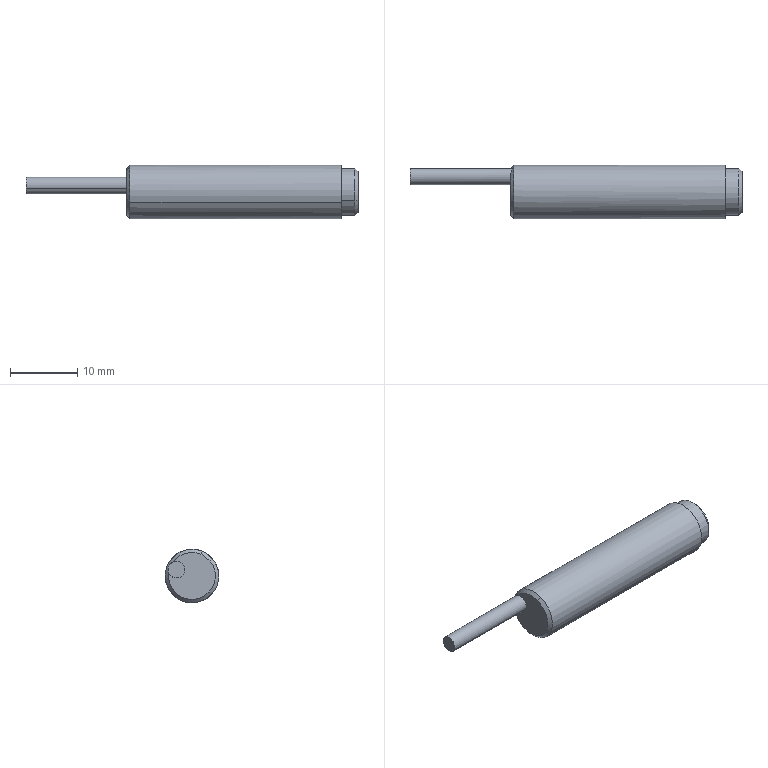Component | SolidWorks | PR8-2DN_1ProximitySwitch-1 | 1 solid | 14 faces | box 49.5 x 8 x 8 mm | volume 1773 mm3 | cylinder 6 | cone 4 | plane 4 | commonest cylinder face diameters 8 x2 7 x2 2.5 x2 | material 45#Steel
STEP:
#1=COLOUR_RGB('',0.7922,0.8196,0.9333);
#2=FILL_AREA_STYLE_COLOUR('',#1);
#3=FILL_AREA_STYLE('',(#2));
#4=SURFACE_STYLE_FILL_AREA(#3);
#5=SURFACE_SIDE_STYLE('',(#4));
#6=SURFACE_STYLE_USAGE(.BOTH.,#5);
#7=PRESENTATION_STYLE_ASSIGNMENT((#6));
#8=CARTESIAN_POINT('',(-0.2322,0.9159,6.515));
#9=VERTEX_POINT('',#8);
#10=CARTESIAN_POINT('',(-0.2322,1.207,6.635));
#11=VERTEX_POINT('',#10);
#12=CARTESIAN_POINT('',(-0.2322,1.061,6.575));
#13=DIRECTION('',(-1.,-0.,-0.));
#14=DIRECTION('',(0.,-0.9245,-0.3811));
#15=AXIS2_PLACEMENT_3D('',#12,#13,#14);
#16=CIRCLE('',#15,0.1575);
#17=EDGE_CURVE('',#9,#11,#16,.T.);
#18=ORIENTED_EDGE('',*,*,#17,.T.);
#19=CARTESIAN_POINT('',(-1.472,1.207,6.635));
#20=VERTEX_POINT('',#19);
#21=CARTESIAN_POINT('',(-0.2322,1.207,6.635));
#22=DIRECTION('',(-1.,-0.,-0.));
#23=VECTOR('',#22,39.37);
#24=LINE('',#21,#23);
#25=EDGE_CURVE('',#11,#20,#24,.T.);
#26=ORIENTED_EDGE('',*,*,#25,.T.);
#27=CARTESIAN_POINT('',(-1.472,1.001,6.72));
#28=VERTEX_POINT('',#27);
#29=CARTESIAN_POINT('',(-1.472,1.061,6.575));
#30=DIRECTION('',(1.,0.,0.));
#31=DIRECTION('',(0.,-0.9245,-0.3811));
#32=AXIS2_PLACEMENT_3D('',#29,#30,#31);
#33=CIRCLE('',#32,0.1575);
#34=EDGE_CURVE('',#20,#28,#33,.T.);
#35=ORIENTED_EDGE('',*,*,#34,.T.);
#36=CARTESIAN_POINT('',(-1.472,0.9159,6.515));
#37=VERTEX_POINT('',#36);
#38=CARTESIAN_POINT('',(-1.472,1.061,6.575));
#39=DIRECTION('',(1.,0.,0.));
#40=DIRECTION('',(0.,-0.9245,-0.3811));
#41=AXIS2_PLACEMENT_3D('',#38,#39,#40);
#42=CIRCLE('',#41,0.1575);
#43=EDGE_CURVE('',#28,#37,#42,.T.);
#44=ORIENTED_EDGE('',*,*,#43,.T.);
#45=CARTESIAN_POINT('',(-0.2322,0.9159,6.515));
#46=DIRECTION('',(-1.,-0.,-0.));
#47=VECTOR('',#46,39.37);
#48=LINE('',#45,#47);
#49=EDGE_CURVE('',#9,#37,#48,.T.);
#50=ORIENTED_EDGE('',*,*,#49,.F.);
#51=EDGE_LOOP('',(#18,#26,#35,#44,#50));
#52=FACE_OUTER_BOUND('',#51,.T.);
#53=CARTESIAN_POINT('',(-0.2322,1.061,6.575));
#54=DIRECTION('',(-1.,-0.,-0.));
#55=DIRECTION('',(0.,-0.9245,-0.3811));
#56=AXIS2_PLACEMENT_3D('',#53,#54,#55);
#57=CYLINDRICAL_SURFACE('',#56,0.1575);
#58=ADVANCED_FACE('',(#52),#57,.T.);
#59=CARTESIAN_POINT('',(-1.492,1.172,6.658));
#60=VERTEX_POINT('',#59);
#61=CARTESIAN_POINT('',(-1.492,1.009,6.702));
#62=VERTEX_POINT('',#61);
#63=CARTESIAN_POINT('',(-1.492,1.061,6.575));
#64=DIRECTION('',(1.,-0.,0.));
#65=DIRECTION('',(0.,0.3811,-0.9245));
#66=AXIS2_PLACEMENT_3D('',#63,#64,#65);
#67=CIRCLE('',#66,0.1378);
#68=EDGE_CURVE('',#60,#62,#67,.T.);
#69=ORIENTED_EDGE('',*,*,#68,.T.);
#70=CARTESIAN_POINT('',(-1.472,1.001,6.72));
#71=DIRECTION('',(0.7071,-0.2695,0.6537));
#72=VECTOR('',#71,39.37);
#73=LINE('',#70,#72);
#74=EDGE_CURVE('',#62,#28,#73,.T.);
#75=ORIENTED_EDGE('',*,*,#74,.T.);
#76=ORIENTED_EDGE('',*,*,#34,.F.);
#77=CARTESIAN_POINT('',(-1.472,1.122,6.429));
#78=VERTEX_POINT('',#77);
#79=CARTESIAN_POINT('',(-1.472,1.061,6.575));
#80=DIRECTION('',(1.,0.,0.));
#81=DIRECTION('',(0.,-0.9245,-0.3811));
#82=AXIS2_PLACEMENT_3D('',#79,#80,#81);
#83=CIRCLE('',#82,0.1575);
#84=EDGE_CURVE('',#78,#20,#83,.T.);
#85=ORIENTED_EDGE('',*,*,#84,.F.);
#86=CARTESIAN_POINT('',(-1.492,1.114,6.447));
#87=VERTEX_POINT('',#86);
#88=CARTESIAN_POINT('',(-1.472,1.122,6.429));
#89=DIRECTION('',(0.7071,0.2695,-0.6537));
#90=VECTOR('',#89,39.37);
#91=LINE('',#88,#90);
#92=EDGE_CURVE('',#87,#78,#91,.T.);
#93=ORIENTED_EDGE('',*,*,#92,.F.);
#94=CARTESIAN_POINT('',(-1.492,1.198,6.594));
#95=VERTEX_POINT('',#94);
#96=CARTESIAN_POINT('',(-1.492,1.061,6.575));
#97=DIRECTION('',(1.,-0.,0.));
#98=DIRECTION('',(0.,0.3811,-0.9245));
#99=AXIS2_PLACEMENT_3D('',#96,#97,#98);
#100=CIRCLE('',#99,0.1378);
#101=EDGE_CURVE('',#87,#95,#100,.T.);
#102=ORIENTED_EDGE('',*,*,#101,.T.);
#103=CARTESIAN_POINT('',(-1.482,1.198,6.631));
#104=VERTEX_POINT('',#103);
#105=CARTESIAN_POINT('',(-1.492,1.198,6.594));
#106=CARTESIAN_POINT('',(-1.491,1.199,6.596));
#107=CARTESIAN_POINT('',(-1.489,1.2,6.599));
#108=CARTESIAN_POINT('',(-1.487,1.201,6.605));
#109=CARTESIAN_POINT('',(-1.486,1.202,6.609));
#110=CARTESIAN_POINT('',(-1.484,1.202,6.615));
#111=CARTESIAN_POINT('',(-1.483,1.201,6.618));
#112=CARTESIAN_POINT('',(-1.482,1.2,6.625));
#113=CARTESIAN_POINT('',(-1.482,1.199,6.628));
#114=CARTESIAN_POINT('',(-1.482,1.198,6.631));
#115=B_SPLINE_CURVE_WITH_KNOTS('',3,(#105,#106,#107,#108,#109,#110,#111,#112,#113,#114),.UNSPECIFIED.,.F.,.F.,(4,2,2,2,4),(0.,0.0002535,0.000507,0.0007605,0.001014),.UNSPECIFIED.);
#116=EDGE_CURVE('',#95,#104,#115,.T.);
#117=ORIENTED_EDGE('',*,*,#116,.T.);
#118=CARTESIAN_POINT('',(-1.482,1.198,6.631));
#119=CARTESIAN_POINT('',(-1.482,1.197,6.634));
#120=CARTESIAN_POINT('',(-1.482,1.195,6.637));
#121=CARTESIAN_POINT('',(-1.483,1.191,6.643));
#122=CARTESIAN_POINT('',(-1.484,1.189,6.645));
#123=CARTESIAN_POINT('',(-1.487,1.182,6.652));
#124=CARTESIAN_POINT('',(-1.489,1.177,6.655));
#125=CARTESIAN_POINT('',(-1.492,1.172,6.658));
#126=B_SPLINE_CURVE_WITH_KNOTS('',3,(#118,#119,#120,#121,#122,#123,#124,#125),.UNSPECIFIED.,.F.,.F.,(4,2,2,4),(0.001014,0.001267,0.001519,0.002025),.UNSPECIFIED.);
#127=EDGE_CURVE('',#104,#60,#126,.T.);
#128=ORIENTED_EDGE('',*,*,#127,.T.);
#129=EDGE_LOOP('',(#69,#75,#76,#85,#93,#102,#117,#128));
#130=FACE_OUTER_BOUND('',#129,.T.);
#131=CARTESIAN_POINT('',(-1.472,1.061,6.575));
#132=DIRECTION('',(1.,-0.,0.));
#133=DIRECTION('',(0.,0.3811,-0.9245));
#134=AXIS2_PLACEMENT_3D('',#131,#132,#133);
#135=CONICAL_SURFACE('',#134,0.1575,0.7854);
#136=ADVANCED_FACE('',(#130),#135,.T.);
#137=CARTESIAN_POINT('',(-0.2322,1.189,6.627));
#138=VERTEX_POINT('',#137);
#139=CARTESIAN_POINT('',(-0.2322,0.9341,6.522));
#140=VERTEX_POINT('',#139);
#141=CARTESIAN_POINT('',(-0.2322,1.061,6.575));
#142=DIRECTION('',(1.,0.,0.));
#143=DIRECTION('',(0.,0.9245,0.3811));
#144=AXIS2_PLACEMENT_3D('',#141,#142,#143);
#145=CIRCLE('',#144,0.1378);
#146=EDGE_CURVE('',#138,#140,#145,.T.);
#147=ORIENTED_EDGE('',*,*,#146,.T.);
#148=CARTESIAN_POINT('',(-0.1534,0.9341,6.522));
#149=VERTEX_POINT('',#148);
#150=CARTESIAN_POINT('',(-0.2322,0.9341,6.522));
#151=DIRECTION('',(1.,0.,0.));
#152=VECTOR('',#151,39.37);
#153=LINE('',#150,#152);
#154=EDGE_CURVE('',#140,#149,#153,.T.);
#155=ORIENTED_EDGE('',*,*,#154,.T.);
#156=CARTESIAN_POINT('',(-0.1534,1.189,6.627));
#157=VERTEX_POINT('',#156);
#158=CARTESIAN_POINT('',(-0.1534,1.061,6.575));
#159=DIRECTION('',(-1.,-0.,-0.));
#160=DIRECTION('',(-0.,0.9245,0.3811));
#161=AXIS2_PLACEMENT_3D('',#158,#159,#160);
#162=CIRCLE('',#161,0.1378);
#163=EDGE_CURVE('',#149,#157,#162,.T.);
#164=ORIENTED_EDGE('',*,*,#163,.T.);
#165=CARTESIAN_POINT('',(-0.2322,1.189,6.627));
#166=DIRECTION('',(1.,0.,0.));
#167=VECTOR('',#166,39.37);
#168=LINE('',#165,#167);
#169=EDGE_CURVE('',#138,#157,#168,.T.);
#170=ORIENTED_EDGE('',*,*,#169,.F.);
#171=EDGE_LOOP('',(#147,#155,#164,#170));
#172=FACE_OUTER_BOUND('',#171,.T.);
#173=CARTESIAN_POINT('',(-0.2322,1.061,6.575));
#174=DIRECTION('',(1.,0.,0.));
#175=DIRECTION('',(0.,0.9245,0.3811));
#176=AXIS2_PLACEMENT_3D('',#173,#174,#175);
#177=CYLINDRICAL_SURFACE('',#176,0.1378);
#178=ADVANCED_FACE('',(#172),#177,.T.);
#179=ORIENTED_EDGE('',*,*,#127,.F.);
#180=CARTESIAN_POINT('',(-2.083,1.198,6.631));
#181=VERTEX_POINT('',#180);
#182=CARTESIAN_POINT('',(-1.492,1.198,6.631));
#183=DIRECTION('',(-1.,-0.,-0.));
#184=VECTOR('',#183,39.37);
#185=LINE('',#182,#184);
#186=EDGE_CURVE('',#104,#181,#185,.T.);
#187=ORIENTED_EDGE('',*,*,#186,.T.);
#188=CARTESIAN_POINT('',(-2.083,1.107,6.594));
#189=VERTEX_POINT('',#188);
#190=CARTESIAN_POINT('',(-2.083,1.152,6.612));
#191=DIRECTION('',(1.,0.,0.));
#192=DIRECTION('',(0.,-0.9245,-0.3811));
#193=AXIS2_PLACEMENT_3D('',#190,#191,#192);
#194=CIRCLE('',#193,0.04921);
#195=EDGE_CURVE('',#181,#189,#194,.T.);
#196=ORIENTED_EDGE('',*,*,#195,.T.);
#197=CARTESIAN_POINT('',(-1.492,1.107,6.594));
#198=VERTEX_POINT('',#197);
#199=CARTESIAN_POINT('',(-1.492,1.107,6.594));
#200=DIRECTION('',(-1.,-0.,-0.));
#201=VECTOR('',#200,39.37);
#202=LINE('',#199,#201);
#203=EDGE_CURVE('',#198,#189,#202,.T.);
#204=ORIENTED_EDGE('',*,*,#203,.F.);
#205=CARTESIAN_POINT('',(-1.492,1.152,6.612));
#206=DIRECTION('',(1.,0.,0.));
#207=DIRECTION('',(0.,-0.9245,-0.3811));
#208=AXIS2_PLACEMENT_3D('',#205,#206,#207);
#209=CIRCLE('',#208,0.04921);
#210=EDGE_CURVE('',#60,#198,#209,.T.);
#211=ORIENTED_EDGE('',*,*,#210,.F.);
#212=EDGE_LOOP('',(#179,#187,#196,#204,#211));
#213=FACE_OUTER_BOUND('',#212,.T.);
#214=CARTESIAN_POINT('',(-1.492,1.152,6.612));
#215=DIRECTION('',(-1.,-0.,-0.));
#216=DIRECTION('',(0.,-0.9245,-0.3811));
#217=AXIS2_PLACEMENT_3D('',#214,#215,#216);
#218=CYLINDRICAL_SURFACE('',#217,0.04921);
#219=ADVANCED_FACE('',(#213),#218,.T.);
#220=CARTESIAN_POINT('',(-0.1338,0.9523,6.53));
#221=VERTEX_POINT('',#220);
#222=CARTESIAN_POINT('',(-0.1338,1.171,6.62));
#223=VERTEX_POINT('',#222);
#224=CARTESIAN_POINT('',(-0.1338,1.061,6.575));
#225=DIRECTION('',(-1.,-0.,-0.));
#226=DIRECTION('',(0.,-0.9245,-0.3811));
#227=AXIS2_PLACEMENT_3D('',#224,#225,#226);
#228=CIRCLE('',#227,0.1181);
#229=EDGE_CURVE('',#221,#223,#228,.T.);
#230=ORIENTED_EDGE('',*,*,#229,.T.);
#231=CARTESIAN_POINT('',(-0.1534,1.189,6.627));
#232=DIRECTION('',(-0.7071,0.6537,0.2695));
#233=VECTOR('',#232,39.37);
#234=LINE('',#231,#233);
#235=EDGE_CURVE('',#223,#157,#234,.T.);
#236=ORIENTED_EDGE('',*,*,#235,.T.);
#237=ORIENTED_EDGE('',*,*,#163,.F.);
#238=CARTESIAN_POINT('',(-0.1534,0.9341,6.522));
#239=DIRECTION('',(-0.7071,-0.6537,-0.2695));
#240=VECTOR('',#239,39.37);
#241=LINE('',#238,#240);
#242=EDGE_CURVE('',#221,#149,#241,.T.);
#243=ORIENTED_EDGE('',*,*,#242,.F.);
#244=EDGE_LOOP('',(#230,#236,#237,#243));
#245=FACE_OUTER_BOUND('',#244,.T.);
#246=CARTESIAN_POINT('',(-0.1534,1.061,6.575));
#247=DIRECTION('',(-1.,-0.,-0.));
#248=DIRECTION('',(0.,-0.9245,-0.3811));
#249=AXIS2_PLACEMENT_3D('',#246,#247,#248);
#250=CONICAL_SURFACE('',#249,0.1378,0.7854);
#251=ADVANCED_FACE('',(#245),#250,.T.);
#252=ORIENTED_EDGE('',*,*,#25,.F.);
#253=CARTESIAN_POINT('',(-0.2322,1.061,6.575));
#254=DIRECTION('',(-1.,-0.,-0.));
#255=DIRECTION('',(0.,-0.9245,-0.3811));
#256=AXIS2_PLACEMENT_3D('',#253,#254,#255);
#257=CIRCLE('',#256,0.1575);
#258=EDGE_CURVE('',#11,#9,#257,.T.);
#259=ORIENTED_EDGE('',*,*,#258,.T.);
#260=ORIENTED_EDGE('',*,*,#49,.T.);
#261=CARTESIAN_POINT('',(-1.472,1.061,6.575));
#262=DIRECTION('',(1.,0.,0.));
#263=DIRECTION('',(0.,-0.9245,-0.3811));
#264=AXIS2_PLACEMENT_3D('',#261,#262,#263);
#265=CIRCLE('',#264,0.1575);
#266=EDGE_CURVE('',#37,#78,#265,.T.);
#267=ORIENTED_EDGE('',*,*,#266,.T.);
#268=ORIENTED_EDGE('',*,*,#84,.T.);
#269=EDGE_LOOP('',(#252,#259,#260,#267,#268));
#270=FACE_OUTER_BOUND('',#269,.T.);
#271=CARTESIAN_POINT('',(-0.2322,1.061,6.575));
#272=DIRECTION('',(-1.,-0.,-0.));
#273=DIRECTION('',(0.,-0.9245,-0.3811));
#274=AXIS2_PLACEMENT_3D('',#271,#272,#273);
#275=CYLINDRICAL_SURFACE('',#274,0.1575);
#276=ADVANCED_FACE('',(#270),#275,.T.);
#277=ORIENTED_EDGE('',*,*,#74,.F.);
#278=CARTESIAN_POINT('',(-1.492,1.061,6.575));
#279=DIRECTION('',(1.,-0.,0.));
#280=DIRECTION('',(0.,0.3811,-0.9245));
#281=AXIS2_PLACEMENT_3D('',#278,#279,#280);
#282=CIRCLE('',#281,0.1378);
#283=EDGE_CURVE('',#62,#87,#282,.T.);
#284=ORIENTED_EDGE('',*,*,#283,.T.);
#285=ORIENTED_EDGE('',*,*,#92,.T.);
#286=ORIENTED_EDGE('',*,*,#266,.F.);
#287=ORIENTED_EDGE('',*,*,#43,.F.);
#288=EDGE_LOOP('',(#277,#284,#285,#286,#287));
#289=FACE_OUTER_BOUND('',#288,.T.);
#290=CARTESIAN_POINT('',(-1.472,1.061,6.575));
#291=DIRECTION('',(1.,-0.,0.));
#292=DIRECTION('',(0.,0.3811,-0.9245));
#293=AXIS2_PLACEMENT_3D('',#290,#291,#292);
#294=CONICAL_SURFACE('',#293,0.1575,0.7854);
#295=ADVANCED_FACE('',(#289),#294,.T.);
#296=ORIENTED_EDGE('',*,*,#146,.F.);
#297=CARTESIAN_POINT('',(-0.2322,1.061,6.575));
#298=DIRECTION('',(1.,0.,0.));
#299=DIRECTION('',(0.,0.9245,0.3811));
#300=AXIS2_PLACEMENT_3D('',#297,#298,#299);
#301=CIRCLE('',#300,0.1378);
#302=EDGE_CURVE('',#140,#138,#301,.T.);
#303=ORIENTED_EDGE('',*,*,#302,.F.);
#304=EDGE_LOOP('',(#296,#303));
#305=FACE_BOUND('',#304,.T.);
#306=ORIENTED_EDGE('',*,*,#17,.F.);
#307=ORIENTED_EDGE('',*,*,#258,.F.);
#308=EDGE_LOOP('',(#306,#307));
#309=FACE_OUTER_BOUND('',#308,.T.);
#310=CARTESIAN_POINT('',(-0.2322,1.061,6.575));
#311=DIRECTION('',(-1.,-0.,-0.));
#312=DIRECTION('',(0.,-0.9245,-0.3811));
#313=AXIS2_PLACEMENT_3D('',#310,#311,#312);
#314=PLANE('',#313);
#315=ADVANCED_FACE('',(#305,#309),#314,.F.);
#316=ORIENTED_EDGE('',*,*,#210,.T.);
#317=CARTESIAN_POINT('',(-1.492,1.152,6.612));
#318=DIRECTION('',(1.,0.,0.));
#319=DIRECTION('',(0.,-0.9245,-0.3811));
#320=AXIS2_PLACEMENT_3D('',#317,#318,#319);
#321=CIRCLE('',#320,0.04921);
#322=EDGE_CURVE('',#198,#95,#321,.T.);
#323=ORIENTED_EDGE('',*,*,#322,.T.);
#324=ORIENTED_EDGE('',*,*,#101,.F.);
#325=ORIENTED_EDGE('',*,*,#283,.F.);
#326=ORIENTED_EDGE('',*,*,#68,.F.);
#327=EDGE_LOOP('',(#316,#323,#324,#325,#326));
#328=FACE_OUTER_BOUND('',#327,.T.);
#329=CARTESIAN_POINT('',(-1.492,1.061,6.575));
#330=DIRECTION('',(-1.,-0.,-0.));
#331=DIRECTION('',(0.,-0.9245,-0.3811));
#332=AXIS2_PLACEMENT_3D('',#329,#330,#331);
#333=PLANE('',#332);
#334=ADVANCED_FACE('',(#328),#333,.T.);
#335=ORIENTED_EDGE('',*,*,#154,.F.);
#336=ORIENTED_EDGE('',*,*,#302,.T.);
#337=ORIENTED_EDGE('',*,*,#169,.T.);
#338=CARTESIAN_POINT('',(-0.1534,1.061,6.575));
#339=DIRECTION('',(-1.,-0.,-0.));
#340=DIRECTION('',(-0.,0.9245,0.3811));
#341=AXIS2_PLACEMENT_3D('',#338,#339,#340);
#342=CIRCLE('',#341,0.1378);
#343=EDGE_CURVE('',#157,#149,#342,.T.);
#344=ORIENTED_EDGE('',*,*,#343,.T.);
#345=EDGE_LOOP('',(#335,#336,#337,#344));
#346=FACE_OUTER_BOUND('',#345,.T.);
#347=CARTESIAN_POINT('',(-0.2322,1.061,6.575));
#348=DIRECTION('',(1.,0.,0.));
#349=DIRECTION('',(0.,0.9245,0.3811));
#350=AXIS2_PLACEMENT_3D('',#347,#348,#349);
#351=CYLINDRICAL_SURFACE('',#350,0.1378);
#352=ADVANCED_FACE('',(#346),#351,.T.);
#353=ORIENTED_EDGE('',*,*,#186,.F.);
#354=ORIENTED_EDGE('',*,*,#116,.F.);
#355=ORIENTED_EDGE('',*,*,#322,.F.);
#356=ORIENTED_EDGE('',*,*,#203,.T.);
#357=CARTESIAN_POINT('',(-2.083,1.152,6.612));
#358=DIRECTION('',(1.,0.,0.));
#359=DIRECTION('',(0.,-0.9245,-0.3811));
#360=AXIS2_PLACEMENT_3D('',#357,#358,#359);
#361=CIRCLE('',#360,0.04921);
#362=EDGE_CURVE('',#189,#181,#361,.T.);
#363=ORIENTED_EDGE('',*,*,#362,.T.);
#364=EDGE_LOOP('',(#353,#354,#355,#356,#363));
#365=FACE_OUTER_BOUND('',#364,.T.);
#366=CARTESIAN_POINT('',(-1.492,1.152,6.612));
#367=DIRECTION('',(-1.,-0.,-0.));
#368=DIRECTION('',(0.,-0.9245,-0.3811));
#369=AXIS2_PLACEMENT_3D('',#366,#367,#368);
#370=CYLINDRICAL_SURFACE('',#369,0.04921);
#371=ADVANCED_FACE('',(#365),#370,.T.);
#372=ORIENTED_EDGE('',*,*,#235,.F.);
#373=CARTESIAN_POINT('',(-0.1338,1.061,6.575));
#374=DIRECTION('',(-1.,-0.,-0.));
#375=DIRECTION('',(0.,-0.9245,-0.3811));
#376=AXIS2_PLACEMENT_3D('',#373,#374,#375);
#377=CIRCLE('',#376,0.1181);
#378=EDGE_CURVE('',#223,#221,#377,.T.);
#379=ORIENTED_EDGE('',*,*,#378,.T.);
#380=ORIENTED_EDGE('',*,*,#242,.T.);
#381=ORIENTED_EDGE('',*,*,#343,.F.);
#382=EDGE_LOOP('',(#372,#379,#380,#381));
#383=FACE_OUTER_BOUND('',#382,.T.);
#384=CARTESIAN_POINT('',(-0.1534,1.061,6.575));
#385=DIRECTION('',(-1.,-0.,-0.));
#386=DIRECTION('',(0.,-0.9245,-0.3811));
#387=AXIS2_PLACEMENT_3D('',#384,#385,#386);
#388=CONICAL_SURFACE('',#387,0.1378,0.7854);
#389=ADVANCED_FACE('',(#383),#388,.T.);
#390=ORIENTED_EDGE('',*,*,#362,.F.);
#391=ORIENTED_EDGE('',*,*,#195,.F.);
#392=EDGE_LOOP('',(#390,#391));
#393=FACE_OUTER_BOUND('',#392,.T.);
#394=CARTESIAN_POINT('',(-2.083,1.061,6.575));
#395=DIRECTION('',(-1.,-0.,-0.));
#396=DIRECTION('',(0.,-0.9245,-0.3811));
#397=AXIS2_PLACEMENT_3D('',#394,#395,#396);
#398=PLANE('',#397);
#399=ADVANCED_FACE('',(#393),#398,.T.);
#400=ORIENTED_EDGE('',*,*,#229,.F.);
#401=ORIENTED_EDGE('',*,*,#378,.F.);
#402=EDGE_LOOP('',(#400,#401));
#403=FACE_OUTER_BOUND('',#402,.T.);
#404=CARTESIAN_POINT('',(-0.1338,1.061,6.575));
#405=DIRECTION('',(1.,0.,0.));
#406=DIRECTION('',(-0.,0.9245,0.3811));
#407=AXIS2_PLACEMENT_3D('',#404,#405,#406);
#408=PLANE('',#407);
#409=ADVANCED_FACE('',(#403),#408,.T.);
#410=CLOSED_SHELL('',(#58,#136,#178,#219,#251,#276,#295,#315,#334,#352,#371,#389,#399,#409));
#411=MANIFOLD_SOLID_BREP('',#410);
#412=STYLED_ITEM('',(#7),#411);
#413=PRESENTATION_LAYER_ASSIGNMENT('','',(#412));
#414=CARTESIAN_POINT('',(0.,0.,0.));
#415=DIRECTION('',(0.,0.,1.));
#416=DIRECTION('',(1.,0.,0.));
#417=AXIS2_PLACEMENT_3D('',#414,#415,#416);
#418=(LENGTH_UNIT()NAMED_UNIT(*)SI_UNIT($,.METRE.));
#419=LENGTH_MEASURE_WITH_UNIT(LENGTH_MEASURE(0.0254),#418);
#420=DIMENSIONAL_EXPONENTS(1.,0.,0.,0.,0.,0.,0.);
#421=(CONVERSION_BASED_UNIT('',#419)LENGTH_UNIT()NAMED_UNIT(#420));
#422=UNCERTAINTY_MEASURE_WITH_UNIT(LENGTH_MEASURE(0.00001),#421,'','');
#423=(NAMED_UNIT(*)PLANE_ANGLE_UNIT()SI_UNIT($,.RADIAN.));
#424=(NAMED_UNIT(*)SI_UNIT($,.STERADIAN.)SOLID_ANGLE_UNIT());
#425=(GEOMETRIC_REPRESENTATION_CONTEXT(3)GLOBAL_UNCERTAINTY_ASSIGNED_CONTEXT((#422))GLOBAL_UNIT_ASSIGNED_CONTEXT((#421,#423,#424))REPRESENTATION_CONTEXT('',''));
#426=ADVANCED_BREP_SHAPE_REPRESENTATION('',(#411,#417),#425);
#427=(LENGTH_UNIT()NAMED_UNIT(*)SI_UNIT($,.METRE.));
#428=LENGTH_MEASURE_WITH_UNIT(LENGTH_MEASURE(0.0254),#427);
#429=DIMENSIONAL_EXPONENTS(1.,0.,0.,0.,0.,0.,0.);
#430=(CONVERSION_BASED_UNIT('',#428)LENGTH_UNIT()NAMED_UNIT(#429));
#431=UNCERTAINTY_MEASURE_WITH_UNIT(LENGTH_MEASURE(0.00001),#430,'','');
#432=(NAMED_UNIT(*)PLANE_ANGLE_UNIT()SI_UNIT($,.RADIAN.));
#433=(NAMED_UNIT(*)SI_UNIT($,.STERADIAN.)SOLID_ANGLE_UNIT());
#434=(GEOMETRIC_REPRESENTATION_CONTEXT(3)GLOBAL_UNCERTAINTY_ASSIGNED_CONTEXT((#431))GLOBAL_UNIT_ASSIGNED_CONTEXT((#430,#432,#433))REPRESENTATION_CONTEXT('',''));
#435=MECHANICAL_DESIGN_GEOMETRIC_PRESENTATION_REPRESENTATION('',(#412),#434);